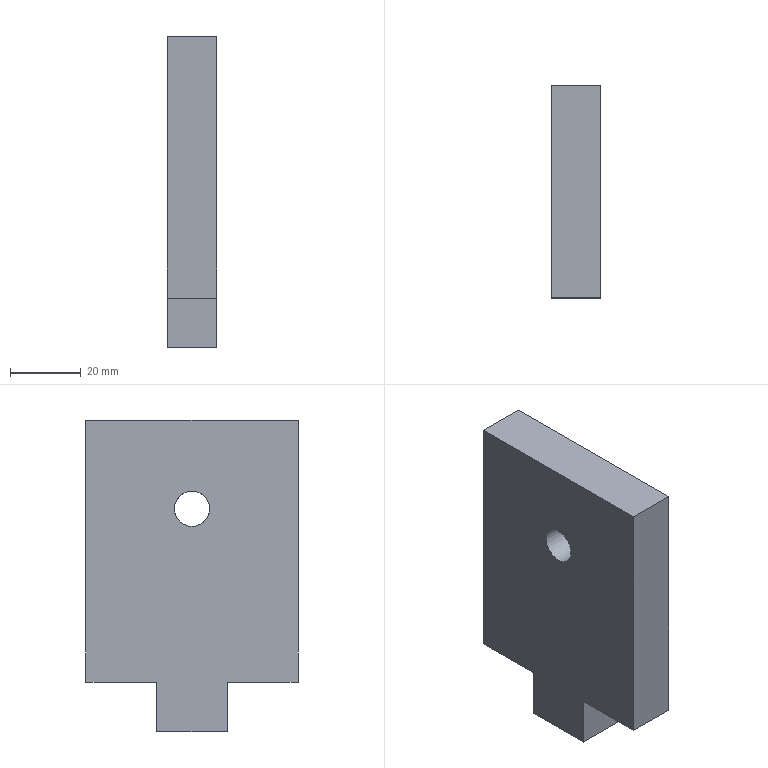Component | NX | 2_VERTICAL_PLATE | 1 solid | 15 faces | box 14 x 60 x 88 mm | volume 64581 mm3 | plane 10 | cylinder 3 | cone 2 | commonest cylinder face diameters 4.2 x2 10 x1
STEP:
#1=CARTESIAN_POINT('',(0.,0.,0.));
#2=DIRECTION('',(0.,0.,1.));
#3=DIRECTION('',(1.,0.,0.));
#4=AXIS2_PLACEMENT_3D('',#1,#2,#3);
#5=CARTESIAN_POINT('',(-0.,-30.,88.));
#6=VERTEX_POINT('',#5);
#7=CARTESIAN_POINT('',(-0.,-30.,14.));
#8=VERTEX_POINT('',#7);
#9=CARTESIAN_POINT('',(-0.,-30.,88.));
#10=DIRECTION('',(0.,0.,-1.));
#11=VECTOR('',#10,1.);
#12=LINE('',#9,#11);
#13=CARTESIAN_POINT('',(14.,-30.,88.));
#14=DIRECTION('',(0.,1.,0.));
#15=DIRECTION('',(0.,-0.,1.));
#16=AXIS2_PLACEMENT_3D('',#13,#14,#15);
#17=PLANE('',#16);
#18=CARTESIAN_POINT('',(0.,-14.));
#19=DIRECTION('',(-1.,0.));
#20=VECTOR('',#19,1.);
#21=LINE('',#18,#20);
#22=(GEOMETRIC_REPRESENTATION_CONTEXT(2)PARAMETRIC_REPRESENTATION_CONTEXT()REPRESENTATION_CONTEXT('',''));
#23=DEFINITIONAL_REPRESENTATION('',(#21),#22);
#24=PCURVE('',#17,#23);
#25=CARTESIAN_POINT('',(-0.,-0.,14.));
#26=DIRECTION('',(1.,0.,0.));
#27=DIRECTION('',(0.,0.,-1.));
#28=AXIS2_PLACEMENT_3D('',#25,#26,#27);
#29=PLANE('',#28);
#30=CARTESIAN_POINT('',(-74.,-30.));
#31=DIRECTION('',(1.,0.));
#32=VECTOR('',#31,1.);
#33=LINE('',#30,#32);
#34=(GEOMETRIC_REPRESENTATION_CONTEXT(2)PARAMETRIC_REPRESENTATION_CONTEXT()REPRESENTATION_CONTEXT('',''));
#35=DEFINITIONAL_REPRESENTATION('',(#33),#34);
#36=PCURVE('',#29,#35);
#37=SURFACE_CURVE('',#12,(#24,#36),.PCURVE_S1.);
#38=EDGE_CURVE('',#6,#8,#37,.T.);
#39=ORIENTED_EDGE('',*,*,#38,.T.);
#40=CARTESIAN_POINT('',(14.,-30.,14.));
#41=VERTEX_POINT('',#40);
#42=CARTESIAN_POINT('',(14.,-30.,14.));
#43=DIRECTION('',(-1.,0.,0.));
#44=VECTOR('',#43,1.);
#45=LINE('',#42,#44);
#46=CARTESIAN_POINT('',(-74.,0.));
#47=DIRECTION('',(0.,-1.));
#48=VECTOR('',#47,1.);
#49=LINE('',#46,#48);
#50=(GEOMETRIC_REPRESENTATION_CONTEXT(2)PARAMETRIC_REPRESENTATION_CONTEXT()REPRESENTATION_CONTEXT('',''));
#51=DEFINITIONAL_REPRESENTATION('',(#49),#50);
#52=PCURVE('',#17,#51);
#53=CARTESIAN_POINT('',(14.,-30.,14.));
#54=DIRECTION('',(0.,0.,1.));
#55=DIRECTION('',(1.,0.,0.));
#56=AXIS2_PLACEMENT_3D('',#53,#54,#55);
#57=PLANE('',#56);
#58=CARTESIAN_POINT('',(0.,0.));
#59=DIRECTION('',(-1.,0.));
#60=VECTOR('',#59,1.);
#61=LINE('',#58,#60);
#62=(GEOMETRIC_REPRESENTATION_CONTEXT(2)PARAMETRIC_REPRESENTATION_CONTEXT()REPRESENTATION_CONTEXT('',''));
#63=DEFINITIONAL_REPRESENTATION('',(#61),#62);
#64=PCURVE('',#57,#63);
#65=SURFACE_CURVE('',#45,(#52,#64),.PCURVE_S1.);
#66=EDGE_CURVE('',#41,#8,#65,.T.);
#67=ORIENTED_EDGE('',*,*,#66,.F.);
#68=CARTESIAN_POINT('',(14.,-30.,88.));
#69=VERTEX_POINT('',#68);
#70=CARTESIAN_POINT('',(14.,-30.,88.));
#71=DIRECTION('',(0.,0.,-1.));
#72=VECTOR('',#71,1.);
#73=LINE('',#70,#72);
#74=CARTESIAN_POINT('',(0.,0.));
#75=DIRECTION('',(-1.,0.));
#76=VECTOR('',#75,1.);
#77=LINE('',#74,#76);
#78=(GEOMETRIC_REPRESENTATION_CONTEXT(2)PARAMETRIC_REPRESENTATION_CONTEXT()REPRESENTATION_CONTEXT('',''));
#79=DEFINITIONAL_REPRESENTATION('',(#77),#78);
#80=PCURVE('',#17,#79);
#81=CARTESIAN_POINT('',(14.,-0.,14.));
#82=DIRECTION('',(1.,0.,0.));
#83=DIRECTION('',(0.,0.,-1.));
#84=AXIS2_PLACEMENT_3D('',#81,#82,#83);
#85=PLANE('',#84);
#86=CARTESIAN_POINT('',(-74.,-30.));
#87=DIRECTION('',(1.,0.));
#88=VECTOR('',#87,1.);
#89=LINE('',#86,#88);
#90=(GEOMETRIC_REPRESENTATION_CONTEXT(2)PARAMETRIC_REPRESENTATION_CONTEXT()REPRESENTATION_CONTEXT('',''));
#91=DEFINITIONAL_REPRESENTATION('',(#89),#90);
#92=PCURVE('',#85,#91);
#93=SURFACE_CURVE('',#73,(#80,#92),.PCURVE_S1.);
#94=EDGE_CURVE('',#69,#41,#93,.T.);
#95=ORIENTED_EDGE('',*,*,#94,.F.);
#96=CARTESIAN_POINT('',(14.,-30.,88.));
#97=DIRECTION('',(-1.,0.,0.));
#98=VECTOR('',#97,1.);
#99=LINE('',#96,#98);
#100=CARTESIAN_POINT('',(0.,0.));
#101=DIRECTION('',(0.,-1.));
#102=VECTOR('',#101,1.);
#103=LINE('',#100,#102);
#104=(GEOMETRIC_REPRESENTATION_CONTEXT(2)PARAMETRIC_REPRESENTATION_CONTEXT()REPRESENTATION_CONTEXT('',''));
#105=DEFINITIONAL_REPRESENTATION('',(#103),#104);
#106=PCURVE('',#17,#105);
#107=CARTESIAN_POINT('',(14.,30.,88.));
#108=DIRECTION('',(0.,0.,-1.));
#109=DIRECTION('',(-1.,0.,0.));
#110=AXIS2_PLACEMENT_3D('',#107,#108,#109);
#111=PLANE('',#110);
#112=CARTESIAN_POINT('',(0.,-60.));
#113=DIRECTION('',(1.,0.));
#114=VECTOR('',#113,1.);
#115=LINE('',#112,#114);
#116=(GEOMETRIC_REPRESENTATION_CONTEXT(2)PARAMETRIC_REPRESENTATION_CONTEXT()REPRESENTATION_CONTEXT('',''));
#117=DEFINITIONAL_REPRESENTATION('',(#115),#116);
#118=PCURVE('',#111,#117);
#119=SURFACE_CURVE('',#99,(#106,#118),.PCURVE_S1.);
#120=EDGE_CURVE('',#69,#6,#119,.T.);
#121=ORIENTED_EDGE('',*,*,#120,.T.);
#122=EDGE_LOOP('',(#39,#67,#95,#121));
#123=FACE_BOUND('',#122,.T.);
#124=ADVANCED_FACE('',(#123),#17,.F.);
#125=CARTESIAN_POINT('',(9.1,-22.,14.));
#126=VERTEX_POINT('',#125);
#127=CARTESIAN_POINT('',(7.,-22.,14.));
#128=DIRECTION('',(0.,0.,1.));
#129=DIRECTION('',(1.,0.,0.));
#130=AXIS2_PLACEMENT_3D('',#127,#128,#129);
#131=CIRCLE('',#130,2.1);
#132=CARTESIAN_POINT('',(-7.,8.));
#133=DIRECTION('',(1.,0.));
#134=AXIS2_PLACEMENT_2D('',#132,#133);
#135=CIRCLE('',#134,2.1);
#136=(GEOMETRIC_REPRESENTATION_CONTEXT(2)PARAMETRIC_REPRESENTATION_CONTEXT()REPRESENTATION_CONTEXT('',''));
#137=DEFINITIONAL_REPRESENTATION('',(#135),#136);
#138=PCURVE('',#57,#137);
#139=CARTESIAN_POINT('',(7.,-22.,14.));
#140=DIRECTION('',(0.,0.,1.));
#141=DIRECTION('',(1.,0.,0.));
#142=AXIS2_PLACEMENT_3D('',#139,#140,#141);
#143=CYLINDRICAL_SURFACE('',#142,2.1);
#144=CARTESIAN_POINT('',(0.,0.));
#145=DIRECTION('',(1.,0.));
#146=VECTOR('',#145,1.);
#147=LINE('',#144,#146);
#148=(GEOMETRIC_REPRESENTATION_CONTEXT(2)PARAMETRIC_REPRESENTATION_CONTEXT()REPRESENTATION_CONTEXT('',''));
#149=DEFINITIONAL_REPRESENTATION('',(#147),#148);
#150=PCURVE('',#143,#149);
#151=SURFACE_CURVE('',#131,(#138,#150),.PCURVE_S1.);
#152=EDGE_CURVE('',#126,#126,#151,.T.);
#153=ORIENTED_EDGE('',*,*,#152,.T.);
#154=EDGE_LOOP('',(#153));
#155=FACE_BOUND('',#154,.T.);
#156=CARTESIAN_POINT('',(-0.,-10.,14.));
#157=VERTEX_POINT('',#156);
#158=CARTESIAN_POINT('',(-0.,-30.,14.));
#159=DIRECTION('',(0.,1.,0.));
#160=VECTOR('',#159,1.);
#161=LINE('',#158,#160);
#162=CARTESIAN_POINT('',(-14.,0.));
#163=DIRECTION('',(0.,1.));
#164=VECTOR('',#163,1.);
#165=LINE('',#162,#164);
#166=(GEOMETRIC_REPRESENTATION_CONTEXT(2)PARAMETRIC_REPRESENTATION_CONTEXT()REPRESENTATION_CONTEXT('',''));
#167=DEFINITIONAL_REPRESENTATION('',(#165),#166);
#168=PCURVE('',#57,#167);
#169=CARTESIAN_POINT('',(0.,-30.));
#170=DIRECTION('',(0.,1.));
#171=VECTOR('',#170,1.);
#172=LINE('',#169,#171);
#173=(GEOMETRIC_REPRESENTATION_CONTEXT(2)PARAMETRIC_REPRESENTATION_CONTEXT()REPRESENTATION_CONTEXT('',''));
#174=DEFINITIONAL_REPRESENTATION('',(#172),#173);
#175=PCURVE('',#29,#174);
#176=SURFACE_CURVE('',#161,(#168,#175),.PCURVE_S1.);
#177=EDGE_CURVE('',#8,#157,#176,.T.);
#178=ORIENTED_EDGE('',*,*,#177,.T.);
#179=CARTESIAN_POINT('',(14.,-10.,14.));
#180=VERTEX_POINT('',#179);
#181=CARTESIAN_POINT('',(14.,-10.,14.));
#182=DIRECTION('',(-1.,0.,0.));
#183=VECTOR('',#182,1.);
#184=LINE('',#181,#183);
#185=CARTESIAN_POINT('',(0.,20.));
#186=DIRECTION('',(-1.,0.));
#187=VECTOR('',#186,1.);
#188=LINE('',#185,#187);
#189=(GEOMETRIC_REPRESENTATION_CONTEXT(2)PARAMETRIC_REPRESENTATION_CONTEXT()REPRESENTATION_CONTEXT('',''));
#190=DEFINITIONAL_REPRESENTATION('',(#188),#189);
#191=PCURVE('',#57,#190);
#192=CARTESIAN_POINT('',(14.,-10.,14.));
#193=DIRECTION('',(0.,1.,0.));
#194=DIRECTION('',(0.,0.,1.));
#195=AXIS2_PLACEMENT_3D('',#192,#193,#194);
#196=PLANE('',#195);
#197=CARTESIAN_POINT('',(0.,0.));
#198=DIRECTION('',(0.,-1.));
#199=VECTOR('',#198,1.);
#200=LINE('',#197,#199);
#201=(GEOMETRIC_REPRESENTATION_CONTEXT(2)PARAMETRIC_REPRESENTATION_CONTEXT()REPRESENTATION_CONTEXT('',''));
#202=DEFINITIONAL_REPRESENTATION('',(#200),#201);
#203=PCURVE('',#196,#202);
#204=SURFACE_CURVE('',#184,(#191,#203),.PCURVE_S1.);
#205=EDGE_CURVE('',#180,#157,#204,.T.);
#206=ORIENTED_EDGE('',*,*,#205,.F.);
#207=CARTESIAN_POINT('',(14.,-30.,14.));
#208=DIRECTION('',(0.,1.,0.));
#209=VECTOR('',#208,1.);
#210=LINE('',#207,#209);
#211=CARTESIAN_POINT('',(0.,0.));
#212=DIRECTION('',(0.,1.));
#213=VECTOR('',#212,1.);
#214=LINE('',#211,#213);
#215=(GEOMETRIC_REPRESENTATION_CONTEXT(2)PARAMETRIC_REPRESENTATION_CONTEXT()REPRESENTATION_CONTEXT('',''));
#216=DEFINITIONAL_REPRESENTATION('',(#214),#215);
#217=PCURVE('',#57,#216);
#218=CARTESIAN_POINT('',(0.,-30.));
#219=DIRECTION('',(0.,1.));
#220=VECTOR('',#219,1.);
#221=LINE('',#218,#220);
#222=(GEOMETRIC_REPRESENTATION_CONTEXT(2)PARAMETRIC_REPRESENTATION_CONTEXT()REPRESENTATION_CONTEXT('',''));
#223=DEFINITIONAL_REPRESENTATION('',(#221),#222);
#224=PCURVE('',#85,#223);
#225=SURFACE_CURVE('',#210,(#217,#224),.PCURVE_S1.);
#226=EDGE_CURVE('',#41,#180,#225,.T.);
#227=ORIENTED_EDGE('',*,*,#226,.F.);
#228=ORIENTED_EDGE('',*,*,#66,.T.);
#229=EDGE_LOOP('',(#178,#206,#227,#228));
#230=FACE_BOUND('',#229,.T.);
#231=ADVANCED_FACE('',(#155,#230),#57,.F.);
#232=CARTESIAN_POINT('',(-0.,-10.,0.));
#233=VERTEX_POINT('',#232);
#234=CARTESIAN_POINT('',(-0.,-10.,14.));
#235=DIRECTION('',(0.,0.,-1.));
#236=VECTOR('',#235,1.);
#237=LINE('',#234,#236);
#238=CARTESIAN_POINT('',(0.,-14.));
#239=DIRECTION('',(-1.,0.));
#240=VECTOR('',#239,1.);
#241=LINE('',#238,#240);
#242=(GEOMETRIC_REPRESENTATION_CONTEXT(2)PARAMETRIC_REPRESENTATION_CONTEXT()REPRESENTATION_CONTEXT('',''));
#243=DEFINITIONAL_REPRESENTATION('',(#241),#242);
#244=PCURVE('',#196,#243);
#245=CARTESIAN_POINT('',(0.,-10.));
#246=DIRECTION('',(1.,0.));
#247=VECTOR('',#246,1.);
#248=LINE('',#245,#247);
#249=(GEOMETRIC_REPRESENTATION_CONTEXT(2)PARAMETRIC_REPRESENTATION_CONTEXT()REPRESENTATION_CONTEXT('',''));
#250=DEFINITIONAL_REPRESENTATION('',(#248),#249);
#251=PCURVE('',#29,#250);
#252=SURFACE_CURVE('',#237,(#244,#251),.PCURVE_S1.);
#253=EDGE_CURVE('',#157,#233,#252,.T.);
#254=ORIENTED_EDGE('',*,*,#253,.T.);
#255=CARTESIAN_POINT('',(14.,-10.,0.));
#256=VERTEX_POINT('',#255);
#257=CARTESIAN_POINT('',(14.,-10.,0.));
#258=DIRECTION('',(-1.,0.,0.));
#259=VECTOR('',#258,1.);
#260=LINE('',#257,#259);
#261=CARTESIAN_POINT('',(-14.,0.));
#262=DIRECTION('',(0.,-1.));
#263=VECTOR('',#262,1.);
#264=LINE('',#261,#263);
#265=(GEOMETRIC_REPRESENTATION_CONTEXT(2)PARAMETRIC_REPRESENTATION_CONTEXT()REPRESENTATION_CONTEXT('',''));
#266=DEFINITIONAL_REPRESENTATION('',(#264),#265);
#267=PCURVE('',#196,#266);
#268=CARTESIAN_POINT('',(14.,-10.,0.));
#269=DIRECTION('',(0.,0.,1.));
#270=DIRECTION('',(1.,0.,0.));
#271=AXIS2_PLACEMENT_3D('',#268,#269,#270);
#272=PLANE('',#271);
#273=CARTESIAN_POINT('',(0.,0.));
#274=DIRECTION('',(-1.,0.));
#275=VECTOR('',#274,1.);
#276=LINE('',#273,#275);
#277=(GEOMETRIC_REPRESENTATION_CONTEXT(2)PARAMETRIC_REPRESENTATION_CONTEXT()REPRESENTATION_CONTEXT('',''));
#278=DEFINITIONAL_REPRESENTATION('',(#276),#277);
#279=PCURVE('',#272,#278);
#280=SURFACE_CURVE('',#260,(#267,#279),.PCURVE_S1.);
#281=EDGE_CURVE('',#256,#233,#280,.T.);
#282=ORIENTED_EDGE('',*,*,#281,.F.);
#283=CARTESIAN_POINT('',(14.,-10.,14.));
#284=DIRECTION('',(0.,0.,-1.));
#285=VECTOR('',#284,1.);
#286=LINE('',#283,#285);
#287=CARTESIAN_POINT('',(0.,0.));
#288=DIRECTION('',(-1.,0.));
#289=VECTOR('',#288,1.);
#290=LINE('',#287,#289);
#291=(GEOMETRIC_REPRESENTATION_CONTEXT(2)PARAMETRIC_REPRESENTATION_CONTEXT()REPRESENTATION_CONTEXT('',''));
#292=DEFINITIONAL_REPRESENTATION('',(#290),#291);
#293=PCURVE('',#196,#292);
#294=CARTESIAN_POINT('',(0.,-10.));
#295=DIRECTION('',(1.,0.));
#296=VECTOR('',#295,1.);
#297=LINE('',#294,#296);
#298=(GEOMETRIC_REPRESENTATION_CONTEXT(2)PARAMETRIC_REPRESENTATION_CONTEXT()REPRESENTATION_CONTEXT('',''));
#299=DEFINITIONAL_REPRESENTATION('',(#297),#298);
#300=PCURVE('',#85,#299);
#301=SURFACE_CURVE('',#286,(#293,#300),.PCURVE_S1.);
#302=EDGE_CURVE('',#180,#256,#301,.T.);
#303=ORIENTED_EDGE('',*,*,#302,.F.);
#304=ORIENTED_EDGE('',*,*,#205,.T.);
#305=EDGE_LOOP('',(#254,#282,#303,#304));
#306=FACE_BOUND('',#305,.T.);
#307=ADVANCED_FACE('',(#306),#196,.F.);
#308=CARTESIAN_POINT('',(-0.,10.,0.));
#309=VERTEX_POINT('',#308);
#310=CARTESIAN_POINT('',(-0.,-10.,0.));
#311=DIRECTION('',(0.,1.,0.));
#312=VECTOR('',#311,1.);
#313=LINE('',#310,#312);
#314=CARTESIAN_POINT('',(-14.,0.));
#315=DIRECTION('',(0.,1.));
#316=VECTOR('',#315,1.);
#317=LINE('',#314,#316);
#318=(GEOMETRIC_REPRESENTATION_CONTEXT(2)PARAMETRIC_REPRESENTATION_CONTEXT()REPRESENTATION_CONTEXT('',''));
#319=DEFINITIONAL_REPRESENTATION('',(#317),#318);
#320=PCURVE('',#272,#319);
#321=CARTESIAN_POINT('',(14.,-10.));
#322=DIRECTION('',(0.,1.));
#323=VECTOR('',#322,1.);
#324=LINE('',#321,#323);
#325=(GEOMETRIC_REPRESENTATION_CONTEXT(2)PARAMETRIC_REPRESENTATION_CONTEXT()REPRESENTATION_CONTEXT('',''));
#326=DEFINITIONAL_REPRESENTATION('',(#324),#325);
#327=PCURVE('',#29,#326);
#328=SURFACE_CURVE('',#313,(#320,#327),.PCURVE_S1.);
#329=EDGE_CURVE('',#233,#309,#328,.T.);
#330=ORIENTED_EDGE('',*,*,#329,.T.);
#331=CARTESIAN_POINT('',(14.,10.,0.));
#332=VERTEX_POINT('',#331);
#333=CARTESIAN_POINT('',(14.,10.,0.));
#334=DIRECTION('',(-1.,0.,0.));
#335=VECTOR('',#334,1.);
#336=LINE('',#333,#335);
#337=CARTESIAN_POINT('',(0.,20.));
#338=DIRECTION('',(-1.,0.));
#339=VECTOR('',#338,1.);
#340=LINE('',#337,#339);
#341=(GEOMETRIC_REPRESENTATION_CONTEXT(2)PARAMETRIC_REPRESENTATION_CONTEXT()REPRESENTATION_CONTEXT('',''));
#342=DEFINITIONAL_REPRESENTATION('',(#340),#341);
#343=PCURVE('',#272,#342);
#344=CARTESIAN_POINT('',(14.,10.,0.));
#345=DIRECTION('',(0.,-1.,-0.));
#346=DIRECTION('',(0.,0.,-1.));
#347=AXIS2_PLACEMENT_3D('',#344,#345,#346);
#348=PLANE('',#347);
#349=CARTESIAN_POINT('',(0.,0.));
#350=DIRECTION('',(0.,-1.));
#351=VECTOR('',#350,1.);
#352=LINE('',#349,#351);
#353=(GEOMETRIC_REPRESENTATION_CONTEXT(2)PARAMETRIC_REPRESENTATION_CONTEXT()REPRESENTATION_CONTEXT('',''));
#354=DEFINITIONAL_REPRESENTATION('',(#352),#353);
#355=PCURVE('',#348,#354);
#356=SURFACE_CURVE('',#336,(#343,#355),.PCURVE_S1.);
#357=EDGE_CURVE('',#332,#309,#356,.T.);
#358=ORIENTED_EDGE('',*,*,#357,.F.);
#359=CARTESIAN_POINT('',(14.,-10.,0.));
#360=DIRECTION('',(0.,1.,0.));
#361=VECTOR('',#360,1.);
#362=LINE('',#359,#361);
#363=CARTESIAN_POINT('',(0.,0.));
#364=DIRECTION('',(0.,1.));
#365=VECTOR('',#364,1.);
#366=LINE('',#363,#365);
#367=(GEOMETRIC_REPRESENTATION_CONTEXT(2)PARAMETRIC_REPRESENTATION_CONTEXT()REPRESENTATION_CONTEXT('',''));
#368=DEFINITIONAL_REPRESENTATION('',(#366),#367);
#369=PCURVE('',#272,#368);
#370=CARTESIAN_POINT('',(14.,-10.));
#371=DIRECTION('',(0.,1.));
#372=VECTOR('',#371,1.);
#373=LINE('',#370,#372);
#374=(GEOMETRIC_REPRESENTATION_CONTEXT(2)PARAMETRIC_REPRESENTATION_CONTEXT()REPRESENTATION_CONTEXT('',''));
#375=DEFINITIONAL_REPRESENTATION('',(#373),#374);
#376=PCURVE('',#85,#375);
#377=SURFACE_CURVE('',#362,(#369,#376),.PCURVE_S1.);
#378=EDGE_CURVE('',#256,#332,#377,.T.);
#379=ORIENTED_EDGE('',*,*,#378,.F.);
#380=ORIENTED_EDGE('',*,*,#281,.T.);
#381=EDGE_LOOP('',(#330,#358,#379,#380));
#382=FACE_BOUND('',#381,.T.);
#383=ADVANCED_FACE('',(#382),#272,.F.);
#384=CARTESIAN_POINT('',(-0.,10.,14.));
#385=VERTEX_POINT('',#384);
#386=CARTESIAN_POINT('',(-0.,10.,0.));
#387=DIRECTION('',(0.,-0.,1.));
#388=VECTOR('',#387,1.);
#389=LINE('',#386,#388);
#390=CARTESIAN_POINT('',(0.,-14.));
#391=DIRECTION('',(-1.,0.));
#392=VECTOR('',#391,1.);
#393=LINE('',#390,#392);
#394=(GEOMETRIC_REPRESENTATION_CONTEXT(2)PARAMETRIC_REPRESENTATION_CONTEXT()REPRESENTATION_CONTEXT('',''));
#395=DEFINITIONAL_REPRESENTATION('',(#393),#394);
#396=PCURVE('',#348,#395);
#397=CARTESIAN_POINT('',(14.,10.));
#398=DIRECTION('',(-1.,-0.));
#399=VECTOR('',#398,1.);
#400=LINE('',#397,#399);
#401=(GEOMETRIC_REPRESENTATION_CONTEXT(2)PARAMETRIC_REPRESENTATION_CONTEXT()REPRESENTATION_CONTEXT('',''));
#402=DEFINITIONAL_REPRESENTATION('',(#400),#401);
#403=PCURVE('',#29,#402);
#404=SURFACE_CURVE('',#389,(#396,#403),.PCURVE_S1.);
#405=EDGE_CURVE('',#309,#385,#404,.T.);
#406=ORIENTED_EDGE('',*,*,#405,.T.);
#407=CARTESIAN_POINT('',(14.,10.,14.));
#408=VERTEX_POINT('',#407);
#409=CARTESIAN_POINT('',(14.,10.,14.));
#410=DIRECTION('',(-1.,0.,0.));
#411=VECTOR('',#410,1.);
#412=LINE('',#409,#411);
#413=CARTESIAN_POINT('',(-14.,0.));
#414=DIRECTION('',(0.,-1.));
#415=VECTOR('',#414,1.);
#416=LINE('',#413,#415);
#417=(GEOMETRIC_REPRESENTATION_CONTEXT(2)PARAMETRIC_REPRESENTATION_CONTEXT()REPRESENTATION_CONTEXT('',''));
#418=DEFINITIONAL_REPRESENTATION('',(#416),#417);
#419=PCURVE('',#348,#418);
#420=CARTESIAN_POINT('',(14.,10.,14.));
#421=DIRECTION('',(0.,0.,1.));
#422=DIRECTION('',(1.,0.,0.));
#423=AXIS2_PLACEMENT_3D('',#420,#421,#422);
#424=PLANE('',#423);
#425=CARTESIAN_POINT('',(0.,0.));
#426=DIRECTION('',(-1.,0.));
#427=VECTOR('',#426,1.);
#428=LINE('',#425,#427);
#429=(GEOMETRIC_REPRESENTATION_CONTEXT(2)PARAMETRIC_REPRESENTATION_CONTEXT()REPRESENTATION_CONTEXT('',''));
#430=DEFINITIONAL_REPRESENTATION('',(#428),#429);
#431=PCURVE('',#424,#430);
#432=SURFACE_CURVE('',#412,(#419,#431),.PCURVE_S1.);
#433=EDGE_CURVE('',#408,#385,#432,.T.);
#434=ORIENTED_EDGE('',*,*,#433,.F.);
#435=CARTESIAN_POINT('',(14.,10.,0.));
#436=DIRECTION('',(0.,-0.,1.));
#437=VECTOR('',#436,1.);
#438=LINE('',#435,#437);
#439=CARTESIAN_POINT('',(0.,0.));
#440=DIRECTION('',(-1.,0.));
#441=VECTOR('',#440,1.);
#442=LINE('',#439,#441);
#443=(GEOMETRIC_REPRESENTATION_CONTEXT(2)PARAMETRIC_REPRESENTATION_CONTEXT()REPRESENTATION_CONTEXT('',''));
#444=DEFINITIONAL_REPRESENTATION('',(#442),#443);
#445=PCURVE('',#348,#444);
#446=CARTESIAN_POINT('',(14.,10.));
#447=DIRECTION('',(-1.,-0.));
#448=VECTOR('',#447,1.);
#449=LINE('',#446,#448);
#450=(GEOMETRIC_REPRESENTATION_CONTEXT(2)PARAMETRIC_REPRESENTATION_CONTEXT()REPRESENTATION_CONTEXT('',''));
#451=DEFINITIONAL_REPRESENTATION('',(#449),#450);
#452=PCURVE('',#85,#451);
#453=SURFACE_CURVE('',#438,(#445,#452),.PCURVE_S1.);
#454=EDGE_CURVE('',#332,#408,#453,.T.);
#455=ORIENTED_EDGE('',*,*,#454,.F.);
#456=ORIENTED_EDGE('',*,*,#357,.T.);
#457=EDGE_LOOP('',(#406,#434,#455,#456));
#458=FACE_BOUND('',#457,.T.);
#459=ADVANCED_FACE('',(#458),#348,.F.);
#460=CARTESIAN_POINT('',(9.1,22.,14.));
#461=VERTEX_POINT('',#460);
#462=CARTESIAN_POINT('',(7.,22.,14.));
#463=DIRECTION('',(0.,0.,1.));
#464=DIRECTION('',(1.,0.,0.));
#465=AXIS2_PLACEMENT_3D('',#462,#463,#464);
#466=CIRCLE('',#465,2.1);
#467=CARTESIAN_POINT('',(-7.,12.));
#468=DIRECTION('',(1.,0.));
#469=AXIS2_PLACEMENT_2D('',#467,#468);
#470=CIRCLE('',#469,2.1);
#471=(GEOMETRIC_REPRESENTATION_CONTEXT(2)PARAMETRIC_REPRESENTATION_CONTEXT()REPRESENTATION_CONTEXT('',''));
#472=DEFINITIONAL_REPRESENTATION('',(#470),#471);
#473=PCURVE('',#424,#472);
#474=CARTESIAN_POINT('',(7.,22.,14.));
#475=DIRECTION('',(0.,0.,1.));
#476=DIRECTION('',(1.,0.,0.));
#477=AXIS2_PLACEMENT_3D('',#474,#475,#476);
#478=CYLINDRICAL_SURFACE('',#477,2.1);
#479=CARTESIAN_POINT('',(0.,0.));
#480=DIRECTION('',(1.,0.));
#481=VECTOR('',#480,1.);
#482=LINE('',#479,#481);
#483=(GEOMETRIC_REPRESENTATION_CONTEXT(2)PARAMETRIC_REPRESENTATION_CONTEXT()REPRESENTATION_CONTEXT('',''));
#484=DEFINITIONAL_REPRESENTATION('',(#482),#483);
#485=PCURVE('',#478,#484);
#486=SURFACE_CURVE('',#466,(#473,#485),.PCURVE_S1.);
#487=EDGE_CURVE('',#461,#461,#486,.T.);
#488=ORIENTED_EDGE('',*,*,#487,.T.);
#489=EDGE_LOOP('',(#488));
#490=FACE_BOUND('',#489,.T.);
#491=CARTESIAN_POINT('',(-0.,30.,14.));
#492=VERTEX_POINT('',#491);
#493=CARTESIAN_POINT('',(-0.,10.,14.));
#494=DIRECTION('',(0.,1.,0.));
#495=VECTOR('',#494,1.);
#496=LINE('',#493,#495);
#497=CARTESIAN_POINT('',(-14.,0.));
#498=DIRECTION('',(0.,1.));
#499=VECTOR('',#498,1.);
#500=LINE('',#497,#499);
#501=(GEOMETRIC_REPRESENTATION_CONTEXT(2)PARAMETRIC_REPRESENTATION_CONTEXT()REPRESENTATION_CONTEXT('',''));
#502=DEFINITIONAL_REPRESENTATION('',(#500),#501);
#503=PCURVE('',#424,#502);
#504=CARTESIAN_POINT('',(0.,10.));
#505=DIRECTION('',(0.,1.));
#506=VECTOR('',#505,1.);
#507=LINE('',#504,#506);
#508=(GEOMETRIC_REPRESENTATION_CONTEXT(2)PARAMETRIC_REPRESENTATION_CONTEXT()REPRESENTATION_CONTEXT('',''));
#509=DEFINITIONAL_REPRESENTATION('',(#507),#508);
#510=PCURVE('',#29,#509);
#511=SURFACE_CURVE('',#496,(#503,#510),.PCURVE_S1.);
#512=EDGE_CURVE('',#385,#492,#511,.T.);
#513=ORIENTED_EDGE('',*,*,#512,.T.);
#514=CARTESIAN_POINT('',(14.,30.,14.));
#515=VERTEX_POINT('',#514);
#516=CARTESIAN_POINT('',(14.,30.,14.));
#517=DIRECTION('',(-1.,0.,0.));
#518=VECTOR('',#517,1.);
#519=LINE('',#516,#518);
#520=CARTESIAN_POINT('',(0.,20.));
#521=DIRECTION('',(-1.,0.));
#522=VECTOR('',#521,1.);
#523=LINE('',#520,#522);
#524=(GEOMETRIC_REPRESENTATION_CONTEXT(2)PARAMETRIC_REPRESENTATION_CONTEXT()REPRESENTATION_CONTEXT('',''));
#525=DEFINITIONAL_REPRESENTATION('',(#523),#524);
#526=PCURVE('',#424,#525);
#527=CARTESIAN_POINT('',(14.,30.,14.));
#528=DIRECTION('',(0.,-1.,0.));
#529=DIRECTION('',(0.,-0.,-1.));
#530=AXIS2_PLACEMENT_3D('',#527,#528,#529);
#531=PLANE('',#530);
#532=CARTESIAN_POINT('',(0.,0.));
#533=DIRECTION('',(0.,-1.));
#534=VECTOR('',#533,1.);
#535=LINE('',#532,#534);
#536=(GEOMETRIC_REPRESENTATION_CONTEXT(2)PARAMETRIC_REPRESENTATION_CONTEXT()REPRESENTATION_CONTEXT('',''));
#537=DEFINITIONAL_REPRESENTATION('',(#535),#536);
#538=PCURVE('',#531,#537);
#539=SURFACE_CURVE('',#519,(#526,#538),.PCURVE_S1.);
#540=EDGE_CURVE('',#515,#492,#539,.T.);
#541=ORIENTED_EDGE('',*,*,#540,.F.);
#542=CARTESIAN_POINT('',(14.,10.,14.));
#543=DIRECTION('',(0.,1.,0.));
#544=VECTOR('',#543,1.);
#545=LINE('',#542,#544);
#546=CARTESIAN_POINT('',(0.,0.));
#547=DIRECTION('',(0.,1.));
#548=VECTOR('',#547,1.);
#549=LINE('',#546,#548);
#550=(GEOMETRIC_REPRESENTATION_CONTEXT(2)PARAMETRIC_REPRESENTATION_CONTEXT()REPRESENTATION_CONTEXT('',''));
#551=DEFINITIONAL_REPRESENTATION('',(#549),#550);
#552=PCURVE('',#424,#551);
#553=CARTESIAN_POINT('',(0.,10.));
#554=DIRECTION('',(0.,1.));
#555=VECTOR('',#554,1.);
#556=LINE('',#553,#555);
#557=(GEOMETRIC_REPRESENTATION_CONTEXT(2)PARAMETRIC_REPRESENTATION_CONTEXT()REPRESENTATION_CONTEXT('',''));
#558=DEFINITIONAL_REPRESENTATION('',(#556),#557);
#559=PCURVE('',#85,#558);
#560=SURFACE_CURVE('',#545,(#552,#559),.PCURVE_S1.);
#561=EDGE_CURVE('',#408,#515,#560,.T.);
#562=ORIENTED_EDGE('',*,*,#561,.F.);
#563=ORIENTED_EDGE('',*,*,#433,.T.);
#564=EDGE_LOOP('',(#513,#541,#562,#563));
#565=FACE_BOUND('',#564,.T.);
#566=ADVANCED_FACE('',(#490,#565),#424,.F.);
#567=CARTESIAN_POINT('',(-0.,30.,88.));
#568=VERTEX_POINT('',#567);
#569=CARTESIAN_POINT('',(-0.,30.,14.));
#570=DIRECTION('',(0.,0.,1.));
#571=VECTOR('',#570,1.);
#572=LINE('',#569,#571);
#573=CARTESIAN_POINT('',(0.,-14.));
#574=DIRECTION('',(-1.,0.));
#575=VECTOR('',#574,1.);
#576=LINE('',#573,#575);
#577=(GEOMETRIC_REPRESENTATION_CONTEXT(2)PARAMETRIC_REPRESENTATION_CONTEXT()REPRESENTATION_CONTEXT('',''));
#578=DEFINITIONAL_REPRESENTATION('',(#576),#577);
#579=PCURVE('',#531,#578);
#580=CARTESIAN_POINT('',(0.,30.));
#581=DIRECTION('',(-1.,0.));
#582=VECTOR('',#581,1.);
#583=LINE('',#580,#582);
#584=(GEOMETRIC_REPRESENTATION_CONTEXT(2)PARAMETRIC_REPRESENTATION_CONTEXT()REPRESENTATION_CONTEXT('',''));
#585=DEFINITIONAL_REPRESENTATION('',(#583),#584);
#586=PCURVE('',#29,#585);
#587=SURFACE_CURVE('',#572,(#579,#586),.PCURVE_S1.);
#588=EDGE_CURVE('',#492,#568,#587,.T.);
#589=ORIENTED_EDGE('',*,*,#588,.T.);
#590=CARTESIAN_POINT('',(14.,30.,88.));
#591=VERTEX_POINT('',#590);
#592=CARTESIAN_POINT('',(14.,30.,88.));
#593=DIRECTION('',(-1.,0.,0.));
#594=VECTOR('',#593,1.);
#595=LINE('',#592,#594);
#596=CARTESIAN_POINT('',(-74.,0.));
#597=DIRECTION('',(0.,-1.));
#598=VECTOR('',#597,1.);
#599=LINE('',#596,#598);
#600=(GEOMETRIC_REPRESENTATION_CONTEXT(2)PARAMETRIC_REPRESENTATION_CONTEXT()REPRESENTATION_CONTEXT('',''));
#601=DEFINITIONAL_REPRESENTATION('',(#599),#600);
#602=PCURVE('',#531,#601);
#603=CARTESIAN_POINT('',(0.,0.));
#604=DIRECTION('',(1.,0.));
#605=VECTOR('',#604,1.);
#606=LINE('',#603,#605);
#607=(GEOMETRIC_REPRESENTATION_CONTEXT(2)PARAMETRIC_REPRESENTATION_CONTEXT()REPRESENTATION_CONTEXT('',''));
#608=DEFINITIONAL_REPRESENTATION('',(#606),#607);
#609=PCURVE('',#111,#608);
#610=SURFACE_CURVE('',#595,(#602,#609),.PCURVE_S1.);
#611=EDGE_CURVE('',#591,#568,#610,.T.);
#612=ORIENTED_EDGE('',*,*,#611,.F.);
#613=CARTESIAN_POINT('',(14.,30.,14.));
#614=DIRECTION('',(0.,0.,1.));
#615=VECTOR('',#614,1.);
#616=LINE('',#613,#615);
#617=CARTESIAN_POINT('',(0.,0.));
#618=DIRECTION('',(-1.,0.));
#619=VECTOR('',#618,1.);
#620=LINE('',#617,#619);
#621=(GEOMETRIC_REPRESENTATION_CONTEXT(2)PARAMETRIC_REPRESENTATION_CONTEXT()REPRESENTATION_CONTEXT('',''));
#622=DEFINITIONAL_REPRESENTATION('',(#620),#621);
#623=PCURVE('',#531,#622);
#624=CARTESIAN_POINT('',(0.,30.));
#625=DIRECTION('',(-1.,0.));
#626=VECTOR('',#625,1.);
#627=LINE('',#624,#626);
#628=(GEOMETRIC_REPRESENTATION_CONTEXT(2)PARAMETRIC_REPRESENTATION_CONTEXT()REPRESENTATION_CONTEXT('',''));
#629=DEFINITIONAL_REPRESENTATION('',(#627),#628);
#630=PCURVE('',#85,#629);
#631=SURFACE_CURVE('',#616,(#623,#630),.PCURVE_S1.);
#632=EDGE_CURVE('',#515,#591,#631,.T.);
#633=ORIENTED_EDGE('',*,*,#632,.F.);
#634=ORIENTED_EDGE('',*,*,#540,.T.);
#635=EDGE_LOOP('',(#589,#612,#633,#634));
#636=FACE_BOUND('',#635,.T.);
#637=ADVANCED_FACE('',(#636),#531,.F.);
#638=CARTESIAN_POINT('',(-0.,30.,88.));
#639=DIRECTION('',(0.,-1.,0.));
#640=VECTOR('',#639,1.);
#641=LINE('',#638,#640);
#642=CARTESIAN_POINT('',(14.,0.));
#643=DIRECTION('',(0.,-1.));
#644=VECTOR('',#643,1.);
#645=LINE('',#642,#644);
#646=(GEOMETRIC_REPRESENTATION_CONTEXT(2)PARAMETRIC_REPRESENTATION_CONTEXT()REPRESENTATION_CONTEXT('',''));
#647=DEFINITIONAL_REPRESENTATION('',(#645),#646);
#648=PCURVE('',#111,#647);
#649=CARTESIAN_POINT('',(-74.,30.));
#650=DIRECTION('',(0.,-1.));
#651=VECTOR('',#650,1.);
#652=LINE('',#649,#651);
#653=(GEOMETRIC_REPRESENTATION_CONTEXT(2)PARAMETRIC_REPRESENTATION_CONTEXT()REPRESENTATION_CONTEXT('',''));
#654=DEFINITIONAL_REPRESENTATION('',(#652),#653);
#655=PCURVE('',#29,#654);
#656=SURFACE_CURVE('',#641,(#648,#655),.PCURVE_S1.);
#657=EDGE_CURVE('',#568,#6,#656,.T.);
#658=ORIENTED_EDGE('',*,*,#657,.T.);
#659=ORIENTED_EDGE('',*,*,#120,.F.);
#660=CARTESIAN_POINT('',(14.,30.,88.));
#661=DIRECTION('',(0.,-1.,0.));
#662=VECTOR('',#661,1.);
#663=LINE('',#660,#662);
#664=CARTESIAN_POINT('',(0.,0.));
#665=DIRECTION('',(0.,-1.));
#666=VECTOR('',#665,1.);
#667=LINE('',#664,#666);
#668=(GEOMETRIC_REPRESENTATION_CONTEXT(2)PARAMETRIC_REPRESENTATION_CONTEXT()REPRESENTATION_CONTEXT('',''));
#669=DEFINITIONAL_REPRESENTATION('',(#667),#668);
#670=PCURVE('',#111,#669);
#671=CARTESIAN_POINT('',(-74.,30.));
#672=DIRECTION('',(0.,-1.));
#673=VECTOR('',#672,1.);
#674=LINE('',#671,#673);
#675=(GEOMETRIC_REPRESENTATION_CONTEXT(2)PARAMETRIC_REPRESENTATION_CONTEXT()REPRESENTATION_CONTEXT('',''));
#676=DEFINITIONAL_REPRESENTATION('',(#674),#675);
#677=PCURVE('',#85,#676);
#678=SURFACE_CURVE('',#663,(#670,#677),.PCURVE_S1.);
#679=EDGE_CURVE('',#591,#69,#678,.T.);
#680=ORIENTED_EDGE('',*,*,#679,.F.);
#681=ORIENTED_EDGE('',*,*,#611,.T.);
#682=EDGE_LOOP('',(#658,#659,#680,#681));
#683=FACE_BOUND('',#682,.T.);
#684=ADVANCED_FACE('',(#683),#111,.F.);
#685=CARTESIAN_POINT('',(14.,5.,63.));
#686=VERTEX_POINT('',#685);
#687=CARTESIAN_POINT('',(14.,-0.,58.));
#688=VERTEX_POINT('',#687);
#689=CARTESIAN_POINT('',(14.,-0.,63.));
#690=DIRECTION('',(1.,0.,0.));
#691=DIRECTION('',(0.,1.,0.));
#692=AXIS2_PLACEMENT_3D('',#689,#690,#691);
#693=CIRCLE('',#692,5.);
#694=CARTESIAN_POINT('',(-49.,0.));
#695=DIRECTION('',(0.,1.));
#696=AXIS2_PLACEMENT_2D('',#694,#695);
#697=CIRCLE('',#696,5.);
#698=(GEOMETRIC_REPRESENTATION_CONTEXT(2)PARAMETRIC_REPRESENTATION_CONTEXT()REPRESENTATION_CONTEXT('',''));
#699=DEFINITIONAL_REPRESENTATION('',(#697),#698);
#700=PCURVE('',#85,#699);
#701=CARTESIAN_POINT('',(-25.,-0.,63.));
#702=DIRECTION('',(1.,0.,0.));
#703=DIRECTION('',(0.,0.,-1.));
#704=AXIS2_PLACEMENT_3D('',#701,#702,#703);
#705=CYLINDRICAL_SURFACE('',#704,5.);
#706=CARTESIAN_POINT('',(1.571,39.));
#707=DIRECTION('',(1.,0.));
#708=VECTOR('',#707,1.);
#709=LINE('',#706,#708);
#710=(GEOMETRIC_REPRESENTATION_CONTEXT(2)PARAMETRIC_REPRESENTATION_CONTEXT()REPRESENTATION_CONTEXT('',''));
#711=DEFINITIONAL_REPRESENTATION('',(#709),#710);
#712=PCURVE('',#705,#711);
#713=SURFACE_CURVE('',#693,(#700,#712),.PCURVE_S1.);
#714=EDGE_CURVE('',#686,#688,#713,.T.);
#715=ORIENTED_EDGE('',*,*,#714,.F.);
#716=CARTESIAN_POINT('',(14.,-0.,63.));
#717=DIRECTION('',(1.,0.,0.));
#718=DIRECTION('',(0.,1.,0.));
#719=AXIS2_PLACEMENT_3D('',#716,#717,#718);
#720=CIRCLE('',#719,5.);
#721=CARTESIAN_POINT('',(-49.,0.));
#722=DIRECTION('',(0.,1.));
#723=AXIS2_PLACEMENT_2D('',#721,#722);
#724=CIRCLE('',#723,5.);
#725=(GEOMETRIC_REPRESENTATION_CONTEXT(2)PARAMETRIC_REPRESENTATION_CONTEXT()REPRESENTATION_CONTEXT('',''));
#726=DEFINITIONAL_REPRESENTATION('',(#724),#725);
#727=PCURVE('',#85,#726);
#728=CARTESIAN_POINT('',(-4.712,39.));
#729=DIRECTION('',(1.,0.));
#730=VECTOR('',#729,1.);
#731=LINE('',#728,#730);
#732=(GEOMETRIC_REPRESENTATION_CONTEXT(2)PARAMETRIC_REPRESENTATION_CONTEXT()REPRESENTATION_CONTEXT('',''));
#733=DEFINITIONAL_REPRESENTATION('',(#731),#732);
#734=PCURVE('',#705,#733);
#735=SURFACE_CURVE('',#720,(#727,#734),.PCURVE_S1.);
#736=EDGE_CURVE('',#688,#686,#735,.T.);
#737=ORIENTED_EDGE('',*,*,#736,.F.);
#738=EDGE_LOOP('',(#715,#737));
#739=FACE_BOUND('',#738,.T.);
#740=ORIENTED_EDGE('',*,*,#94,.T.);
#741=ORIENTED_EDGE('',*,*,#226,.T.);
#742=ORIENTED_EDGE('',*,*,#302,.T.);
#743=ORIENTED_EDGE('',*,*,#378,.T.);
#744=ORIENTED_EDGE('',*,*,#454,.T.);
#745=ORIENTED_EDGE('',*,*,#561,.T.);
#746=ORIENTED_EDGE('',*,*,#632,.T.);
#747=ORIENTED_EDGE('',*,*,#679,.T.);
#748=EDGE_LOOP('',(#740,#741,#742,#743,#744,#745,#746,#747));
#749=FACE_BOUND('',#748,.T.);
#750=ADVANCED_FACE('',(#739,#749),#85,.T.);
#751=CARTESIAN_POINT('',(-0.,-0.,58.));
#752=VERTEX_POINT('',#751);
#753=CARTESIAN_POINT('',(-0.,-0.,63.));
#754=DIRECTION('',(1.,0.,0.));
#755=DIRECTION('',(0.,0.,-1.));
#756=AXIS2_PLACEMENT_3D('',#753,#754,#755);
#757=CIRCLE('',#756,5.);
#758=CARTESIAN_POINT('',(-49.,0.));
#759=DIRECTION('',(1.,0.));
#760=AXIS2_PLACEMENT_2D('',#758,#759);
#761=CIRCLE('',#760,5.);
#762=(GEOMETRIC_REPRESENTATION_CONTEXT(2)PARAMETRIC_REPRESENTATION_CONTEXT()REPRESENTATION_CONTEXT('',''));
#763=DEFINITIONAL_REPRESENTATION('',(#761),#762);
#764=PCURVE('',#29,#763);
#765=CARTESIAN_POINT('',(0.,25.));
#766=DIRECTION('',(1.,0.));
#767=VECTOR('',#766,1.);
#768=LINE('',#765,#767);
#769=(GEOMETRIC_REPRESENTATION_CONTEXT(2)PARAMETRIC_REPRESENTATION_CONTEXT()REPRESENTATION_CONTEXT('',''));
#770=DEFINITIONAL_REPRESENTATION('',(#768),#769);
#771=PCURVE('',#705,#770);
#772=SURFACE_CURVE('',#757,(#764,#771),.PCURVE_S1.);
#773=EDGE_CURVE('',#752,#752,#772,.T.);
#774=ORIENTED_EDGE('',*,*,#773,.T.);
#775=EDGE_LOOP('',(#774));
#776=FACE_BOUND('',#775,.T.);
#777=ORIENTED_EDGE('',*,*,#38,.F.);
#778=ORIENTED_EDGE('',*,*,#657,.F.);
#779=ORIENTED_EDGE('',*,*,#588,.F.);
#780=ORIENTED_EDGE('',*,*,#512,.F.);
#781=ORIENTED_EDGE('',*,*,#405,.F.);
#782=ORIENTED_EDGE('',*,*,#329,.F.);
#783=ORIENTED_EDGE('',*,*,#253,.F.);
#784=ORIENTED_EDGE('',*,*,#177,.F.);
#785=EDGE_LOOP('',(#777,#778,#779,#780,#781,#782,#783,#784));
#786=FACE_BOUND('',#785,.T.);
#787=ADVANCED_FACE('',(#776,#786),#29,.F.);
#788=ORIENTED_EDGE('',*,*,#736,.F.);
#789=CARTESIAN_POINT('',(-0.,-0.,58.));
#790=CARTESIAN_POINT('',(14.,-0.,58.));
#791=B_SPLINE_CURVE_WITH_KNOTS('',1,(#789,#790),.UNSPECIFIED.,.F.,.F.,(2,2),(25.,39.),.PIECEWISE_BEZIER_KNOTS.);
#792=CARTESIAN_POINT('',(0.,0.));
#793=DIRECTION('',(0.,1.));
#794=VECTOR('',#793,1.);
#795=LINE('',#792,#794);
#796=(GEOMETRIC_REPRESENTATION_CONTEXT(2)PARAMETRIC_REPRESENTATION_CONTEXT()REPRESENTATION_CONTEXT('',''));
#797=DEFINITIONAL_REPRESENTATION('',(#795),#796);
#798=PCURVE('',#705,#797);
#799=CARTESIAN_POINT('',(6.283,0.));
#800=DIRECTION('',(0.,1.));
#801=VECTOR('',#800,1.);
#802=LINE('',#799,#801);
#803=(GEOMETRIC_REPRESENTATION_CONTEXT(2)PARAMETRIC_REPRESENTATION_CONTEXT()REPRESENTATION_CONTEXT('',''));
#804=DEFINITIONAL_REPRESENTATION('',(#802),#803);
#805=PCURVE('',#705,#804);
#806=SEAM_CURVE('',#791,(#798,#805),.PCURVE_S1.);
#807=EDGE_CURVE('',#752,#688,#806,.T.);
#808=ORIENTED_EDGE('',*,*,#807,.F.);
#809=ORIENTED_EDGE('',*,*,#773,.T.);
#810=ORIENTED_EDGE('',*,*,#807,.T.);
#811=ORIENTED_EDGE('',*,*,#714,.F.);
#812=EDGE_LOOP('',(#788,#808,#809,#810,#811));
#813=FACE_BOUND('',#812,.F.);
#814=ADVANCED_FACE('',(#813),#705,.F.);
#815=CARTESIAN_POINT('',(4.9,-22.,28.));
#816=VERTEX_POINT('',#815);
#817=CARTESIAN_POINT('',(9.1,-22.,28.));
#818=VERTEX_POINT('',#817);
#819=CARTESIAN_POINT('',(7.,-22.,28.));
#820=DIRECTION('',(0.,0.,-1.));
#821=DIRECTION('',(1.,0.,0.));
#822=AXIS2_PLACEMENT_3D('',#819,#820,#821);
#823=CIRCLE('',#822,2.1);
#824=CARTESIAN_POINT('',(7.,-22.,28.));
#825=DIRECTION('',(0.,0.,-1.));
#826=DIRECTION('',(-1.,0.,0.));
#827=AXIS2_PLACEMENT_3D('',#824,#825,#826);
#828=CONICAL_SURFACE('',#827,2.1,1.03);
#829=CARTESIAN_POINT('',(-3.142,0.));
#830=DIRECTION('',(1.,0.));
#831=VECTOR('',#830,1.);
#832=LINE('',#829,#831);
#833=(GEOMETRIC_REPRESENTATION_CONTEXT(2)PARAMETRIC_REPRESENTATION_CONTEXT()REPRESENTATION_CONTEXT('',''));
#834=DEFINITIONAL_REPRESENTATION('',(#832),#833);
#835=PCURVE('',#828,#834);
#836=CARTESIAN_POINT('',(6.283,14.));
#837=DIRECTION('',(-1.,0.));
#838=VECTOR('',#837,1.);
#839=LINE('',#836,#838);
#840=(GEOMETRIC_REPRESENTATION_CONTEXT(2)PARAMETRIC_REPRESENTATION_CONTEXT()REPRESENTATION_CONTEXT('',''));
#841=DEFINITIONAL_REPRESENTATION('',(#839),#840);
#842=PCURVE('',#143,#841);
#843=SURFACE_CURVE('',#823,(#835,#842),.PCURVE_S1.);
#844=EDGE_CURVE('',#816,#818,#843,.T.);
#845=ORIENTED_EDGE('',*,*,#844,.F.);
#846=CARTESIAN_POINT('',(7.,-22.,29.262));
#847=VERTEX_POINT('',#846);
#848=CARTESIAN_POINT('',(7.,-22.,29.262));
#849=CARTESIAN_POINT('',(4.9,-22.,28.));
#850=B_SPLINE_CURVE_WITH_KNOTS('',1,(#848,#849),.UNSPECIFIED.,.F.,.F.,(2,2),(-2.45,0.),.PIECEWISE_BEZIER_KNOTS.);
#851=CARTESIAN_POINT('',(0.,0.));
#852=DIRECTION('',(0.,1.));
#853=VECTOR('',#852,1.);
#854=LINE('',#851,#853);
#855=(GEOMETRIC_REPRESENTATION_CONTEXT(2)PARAMETRIC_REPRESENTATION_CONTEXT()REPRESENTATION_CONTEXT('',''));
#856=DEFINITIONAL_REPRESENTATION('',(#854),#855);
#857=PCURVE('',#828,#856);
#858=CARTESIAN_POINT('',(6.283,0.));
#859=DIRECTION('',(0.,1.));
#860=VECTOR('',#859,1.);
#861=LINE('',#858,#860);
#862=(GEOMETRIC_REPRESENTATION_CONTEXT(2)PARAMETRIC_REPRESENTATION_CONTEXT()REPRESENTATION_CONTEXT('',''));
#863=DEFINITIONAL_REPRESENTATION('',(#861),#862);
#864=PCURVE('',#828,#863);
#865=SEAM_CURVE('',#850,(#857,#864),.PCURVE_S1.);
#866=EDGE_CURVE('',#847,#816,#865,.T.);
#867=ORIENTED_EDGE('',*,*,#866,.F.);
#868=ORIENTED_EDGE('',*,*,#866,.T.);
#869=CARTESIAN_POINT('',(7.,-22.,28.));
#870=DIRECTION('',(0.,0.,-1.));
#871=DIRECTION('',(1.,0.,0.));
#872=AXIS2_PLACEMENT_3D('',#869,#870,#871);
#873=CIRCLE('',#872,2.1);
#874=CARTESIAN_POINT('',(3.142,0.));
#875=DIRECTION('',(1.,0.));
#876=VECTOR('',#875,1.);
#877=LINE('',#874,#876);
#878=(GEOMETRIC_REPRESENTATION_CONTEXT(2)PARAMETRIC_REPRESENTATION_CONTEXT()REPRESENTATION_CONTEXT('',''));
#879=DEFINITIONAL_REPRESENTATION('',(#877),#878);
#880=PCURVE('',#828,#879);
#881=CARTESIAN_POINT('',(6.283,14.));
#882=DIRECTION('',(-1.,0.));
#883=VECTOR('',#882,1.);
#884=LINE('',#881,#883);
#885=(GEOMETRIC_REPRESENTATION_CONTEXT(2)PARAMETRIC_REPRESENTATION_CONTEXT()REPRESENTATION_CONTEXT('',''));
#886=DEFINITIONAL_REPRESENTATION('',(#884),#885);
#887=PCURVE('',#143,#886);
#888=SURFACE_CURVE('',#873,(#880,#887),.PCURVE_S1.);
#889=EDGE_CURVE('',#818,#816,#888,.T.);
#890=ORIENTED_EDGE('',*,*,#889,.F.);
#891=EDGE_LOOP('',(#845,#867,#868,#890));
#892=FACE_BOUND('',#891,.F.);
#893=ADVANCED_FACE('',(#892),#828,.F.);
#894=ORIENTED_EDGE('',*,*,#844,.T.);
#895=CARTESIAN_POINT('',(9.1,-22.,14.));
#896=CARTESIAN_POINT('',(9.1,-22.,28.));
#897=B_SPLINE_CURVE_WITH_KNOTS('',1,(#895,#896),.UNSPECIFIED.,.F.,.F.,(2,2),(0.,14.),.PIECEWISE_BEZIER_KNOTS.);
#898=CARTESIAN_POINT('',(0.,0.));
#899=DIRECTION('',(0.,1.));
#900=VECTOR('',#899,1.);
#901=LINE('',#898,#900);
#902=(GEOMETRIC_REPRESENTATION_CONTEXT(2)PARAMETRIC_REPRESENTATION_CONTEXT()REPRESENTATION_CONTEXT('',''));
#903=DEFINITIONAL_REPRESENTATION('',(#901),#902);
#904=PCURVE('',#143,#903);
#905=CARTESIAN_POINT('',(6.283,0.));
#906=DIRECTION('',(0.,1.));
#907=VECTOR('',#906,1.);
#908=LINE('',#905,#907);
#909=(GEOMETRIC_REPRESENTATION_CONTEXT(2)PARAMETRIC_REPRESENTATION_CONTEXT()REPRESENTATION_CONTEXT('',''));
#910=DEFINITIONAL_REPRESENTATION('',(#908),#909);
#911=PCURVE('',#143,#910);
#912=SEAM_CURVE('',#897,(#904,#911),.PCURVE_S1.);
#913=EDGE_CURVE('',#126,#818,#912,.T.);
#914=ORIENTED_EDGE('',*,*,#913,.F.);
#915=ORIENTED_EDGE('',*,*,#152,.T.);
#916=ORIENTED_EDGE('',*,*,#913,.T.);
#917=ORIENTED_EDGE('',*,*,#889,.T.);
#918=EDGE_LOOP('',(#894,#914,#915,#916,#917));
#919=FACE_BOUND('',#918,.F.);
#920=ADVANCED_FACE('',(#919),#143,.F.);
#921=CARTESIAN_POINT('',(4.9,22.,28.));
#922=VERTEX_POINT('',#921);
#923=CARTESIAN_POINT('',(9.1,22.,28.));
#924=VERTEX_POINT('',#923);
#925=CARTESIAN_POINT('',(7.,22.,28.));
#926=DIRECTION('',(0.,0.,-1.));
#927=DIRECTION('',(1.,0.,0.));
#928=AXIS2_PLACEMENT_3D('',#925,#926,#927);
#929=CIRCLE('',#928,2.1);
#930=CARTESIAN_POINT('',(7.,22.,28.));
#931=DIRECTION('',(0.,0.,-1.));
#932=DIRECTION('',(-1.,0.,0.));
#933=AXIS2_PLACEMENT_3D('',#930,#931,#932);
#934=CONICAL_SURFACE('',#933,2.1,1.03);
#935=CARTESIAN_POINT('',(-3.142,0.));
#936=DIRECTION('',(1.,0.));
#937=VECTOR('',#936,1.);
#938=LINE('',#935,#937);
#939=(GEOMETRIC_REPRESENTATION_CONTEXT(2)PARAMETRIC_REPRESENTATION_CONTEXT()REPRESENTATION_CONTEXT('',''));
#940=DEFINITIONAL_REPRESENTATION('',(#938),#939);
#941=PCURVE('',#934,#940);
#942=CARTESIAN_POINT('',(6.283,14.));
#943=DIRECTION('',(-1.,0.));
#944=VECTOR('',#943,1.);
#945=LINE('',#942,#944);
#946=(GEOMETRIC_REPRESENTATION_CONTEXT(2)PARAMETRIC_REPRESENTATION_CONTEXT()REPRESENTATION_CONTEXT('',''));
#947=DEFINITIONAL_REPRESENTATION('',(#945),#946);
#948=PCURVE('',#478,#947);
#949=SURFACE_CURVE('',#929,(#941,#948),.PCURVE_S1.);
#950=EDGE_CURVE('',#922,#924,#949,.T.);
#951=ORIENTED_EDGE('',*,*,#950,.F.);
#952=CARTESIAN_POINT('',(7.,22.,29.262));
#953=VERTEX_POINT('',#952);
#954=CARTESIAN_POINT('',(7.,22.,29.262));
#955=CARTESIAN_POINT('',(4.9,22.,28.));
#956=B_SPLINE_CURVE_WITH_KNOTS('',1,(#954,#955),.UNSPECIFIED.,.F.,.F.,(2,2),(-2.45,0.),.PIECEWISE_BEZIER_KNOTS.);
#957=CARTESIAN_POINT('',(0.,0.));
#958=DIRECTION('',(0.,1.));
#959=VECTOR('',#958,1.);
#960=LINE('',#957,#959);
#961=(GEOMETRIC_REPRESENTATION_CONTEXT(2)PARAMETRIC_REPRESENTATION_CONTEXT()REPRESENTATION_CONTEXT('',''));
#962=DEFINITIONAL_REPRESENTATION('',(#960),#961);
#963=PCURVE('',#934,#962);
#964=CARTESIAN_POINT('',(6.283,0.));
#965=DIRECTION('',(0.,1.));
#966=VECTOR('',#965,1.);
#967=LINE('',#964,#966);
#968=(GEOMETRIC_REPRESENTATION_CONTEXT(2)PARAMETRIC_REPRESENTATION_CONTEXT()REPRESENTATION_CONTEXT('',''));
#969=DEFINITIONAL_REPRESENTATION('',(#967),#968);
#970=PCURVE('',#934,#969);
#971=SEAM_CURVE('',#956,(#963,#970),.PCURVE_S1.);
#972=EDGE_CURVE('',#953,#922,#971,.T.);
#973=ORIENTED_EDGE('',*,*,#972,.F.);
#974=ORIENTED_EDGE('',*,*,#972,.T.);
#975=CARTESIAN_POINT('',(7.,22.,28.));
#976=DIRECTION('',(0.,0.,-1.));
#977=DIRECTION('',(1.,0.,0.));
#978=AXIS2_PLACEMENT_3D('',#975,#976,#977);
#979=CIRCLE('',#978,2.1);
#980=CARTESIAN_POINT('',(3.142,0.));
#981=DIRECTION('',(1.,0.));
#982=VECTOR('',#981,1.);
#983=LINE('',#980,#982);
#984=(GEOMETRIC_REPRESENTATION_CONTEXT(2)PARAMETRIC_REPRESENTATION_CONTEXT()REPRESENTATION_CONTEXT('',''));
#985=DEFINITIONAL_REPRESENTATION('',(#983),#984);
#986=PCURVE('',#934,#985);
#987=CARTESIAN_POINT('',(6.283,14.));
#988=DIRECTION('',(-1.,0.));
#989=VECTOR('',#988,1.);
#990=LINE('',#987,#989);
#991=(GEOMETRIC_REPRESENTATION_CONTEXT(2)PARAMETRIC_REPRESENTATION_CONTEXT()REPRESENTATION_CONTEXT('',''));
#992=DEFINITIONAL_REPRESENTATION('',(#990),#991);
#993=PCURVE('',#478,#992);
#994=SURFACE_CURVE('',#979,(#986,#993),.PCURVE_S1.);
#995=EDGE_CURVE('',#924,#922,#994,.T.);
#996=ORIENTED_EDGE('',*,*,#995,.F.);
#997=EDGE_LOOP('',(#951,#973,#974,#996));
#998=FACE_BOUND('',#997,.F.);
#999=ADVANCED_FACE('',(#998),#934,.F.);
#1000=ORIENTED_EDGE('',*,*,#950,.T.);
#1001=CARTESIAN_POINT('',(9.1,22.,14.));
#1002=CARTESIAN_POINT('',(9.1,22.,28.));
#1003=B_SPLINE_CURVE_WITH_KNOTS('',1,(#1001,#1002),.UNSPECIFIED.,.F.,.F.,(2,2),(0.,14.),.PIECEWISE_BEZIER_KNOTS.);
#1004=CARTESIAN_POINT('',(0.,0.));
#1005=DIRECTION('',(0.,1.));
#1006=VECTOR('',#1005,1.);
#1007=LINE('',#1004,#1006);
#1008=(GEOMETRIC_REPRESENTATION_CONTEXT(2)PARAMETRIC_REPRESENTATION_CONTEXT()REPRESENTATION_CONTEXT('',''));
#1009=DEFINITIONAL_REPRESENTATION('',(#1007),#1008);
#1010=PCURVE('',#478,#1009);
#1011=CARTESIAN_POINT('',(6.283,0.));
#1012=DIRECTION('',(0.,1.));
#1013=VECTOR('',#1012,1.);
#1014=LINE('',#1011,#1013);
#1015=(GEOMETRIC_REPRESENTATION_CONTEXT(2)PARAMETRIC_REPRESENTATION_CONTEXT()REPRESENTATION_CONTEXT('',''));
#1016=DEFINITIONAL_REPRESENTATION('',(#1014),#1015);
#1017=PCURVE('',#478,#1016);
#1018=SEAM_CURVE('',#1003,(#1010,#1017),.PCURVE_S1.);
#1019=EDGE_CURVE('',#461,#924,#1018,.T.);
#1020=ORIENTED_EDGE('',*,*,#1019,.F.);
#1021=ORIENTED_EDGE('',*,*,#487,.T.);
#1022=ORIENTED_EDGE('',*,*,#1019,.T.);
#1023=ORIENTED_EDGE('',*,*,#995,.T.);
#1024=EDGE_LOOP('',(#1000,#1020,#1021,#1022,#1023));
#1025=FACE_BOUND('',#1024,.F.);
#1026=ADVANCED_FACE('',(#1025),#478,.F.);
#1027=CLOSED_SHELL('',(#124,#231,#307,#383,#459,#566,#637,#684,#750,#787,#814,#893,#920,#999,#1026));
#1028=MANIFOLD_SOLID_BREP('',#1027);
#1029=(LENGTH_UNIT()NAMED_UNIT(*)SI_UNIT(.MILLI.,.METRE.));
#1030=UNCERTAINTY_MEASURE_WITH_UNIT(LENGTH_MEASURE(0.000002),#1029,'','');
#1031=(NAMED_UNIT(*)PLANE_ANGLE_UNIT()SI_UNIT($,.RADIAN.));
#1032=(NAMED_UNIT(*)SI_UNIT($,.STERADIAN.)SOLID_ANGLE_UNIT());
#1033=(GEOMETRIC_REPRESENTATION_CONTEXT(3)GLOBAL_UNCERTAINTY_ASSIGNED_CONTEXT((#1030))GLOBAL_UNIT_ASSIGNED_CONTEXT((#1029,#1031,#1032))REPRESENTATION_CONTEXT('',''));
#1034=ADVANCED_BREP_SHAPE_REPRESENTATION('',(#4,#1028),#1033);